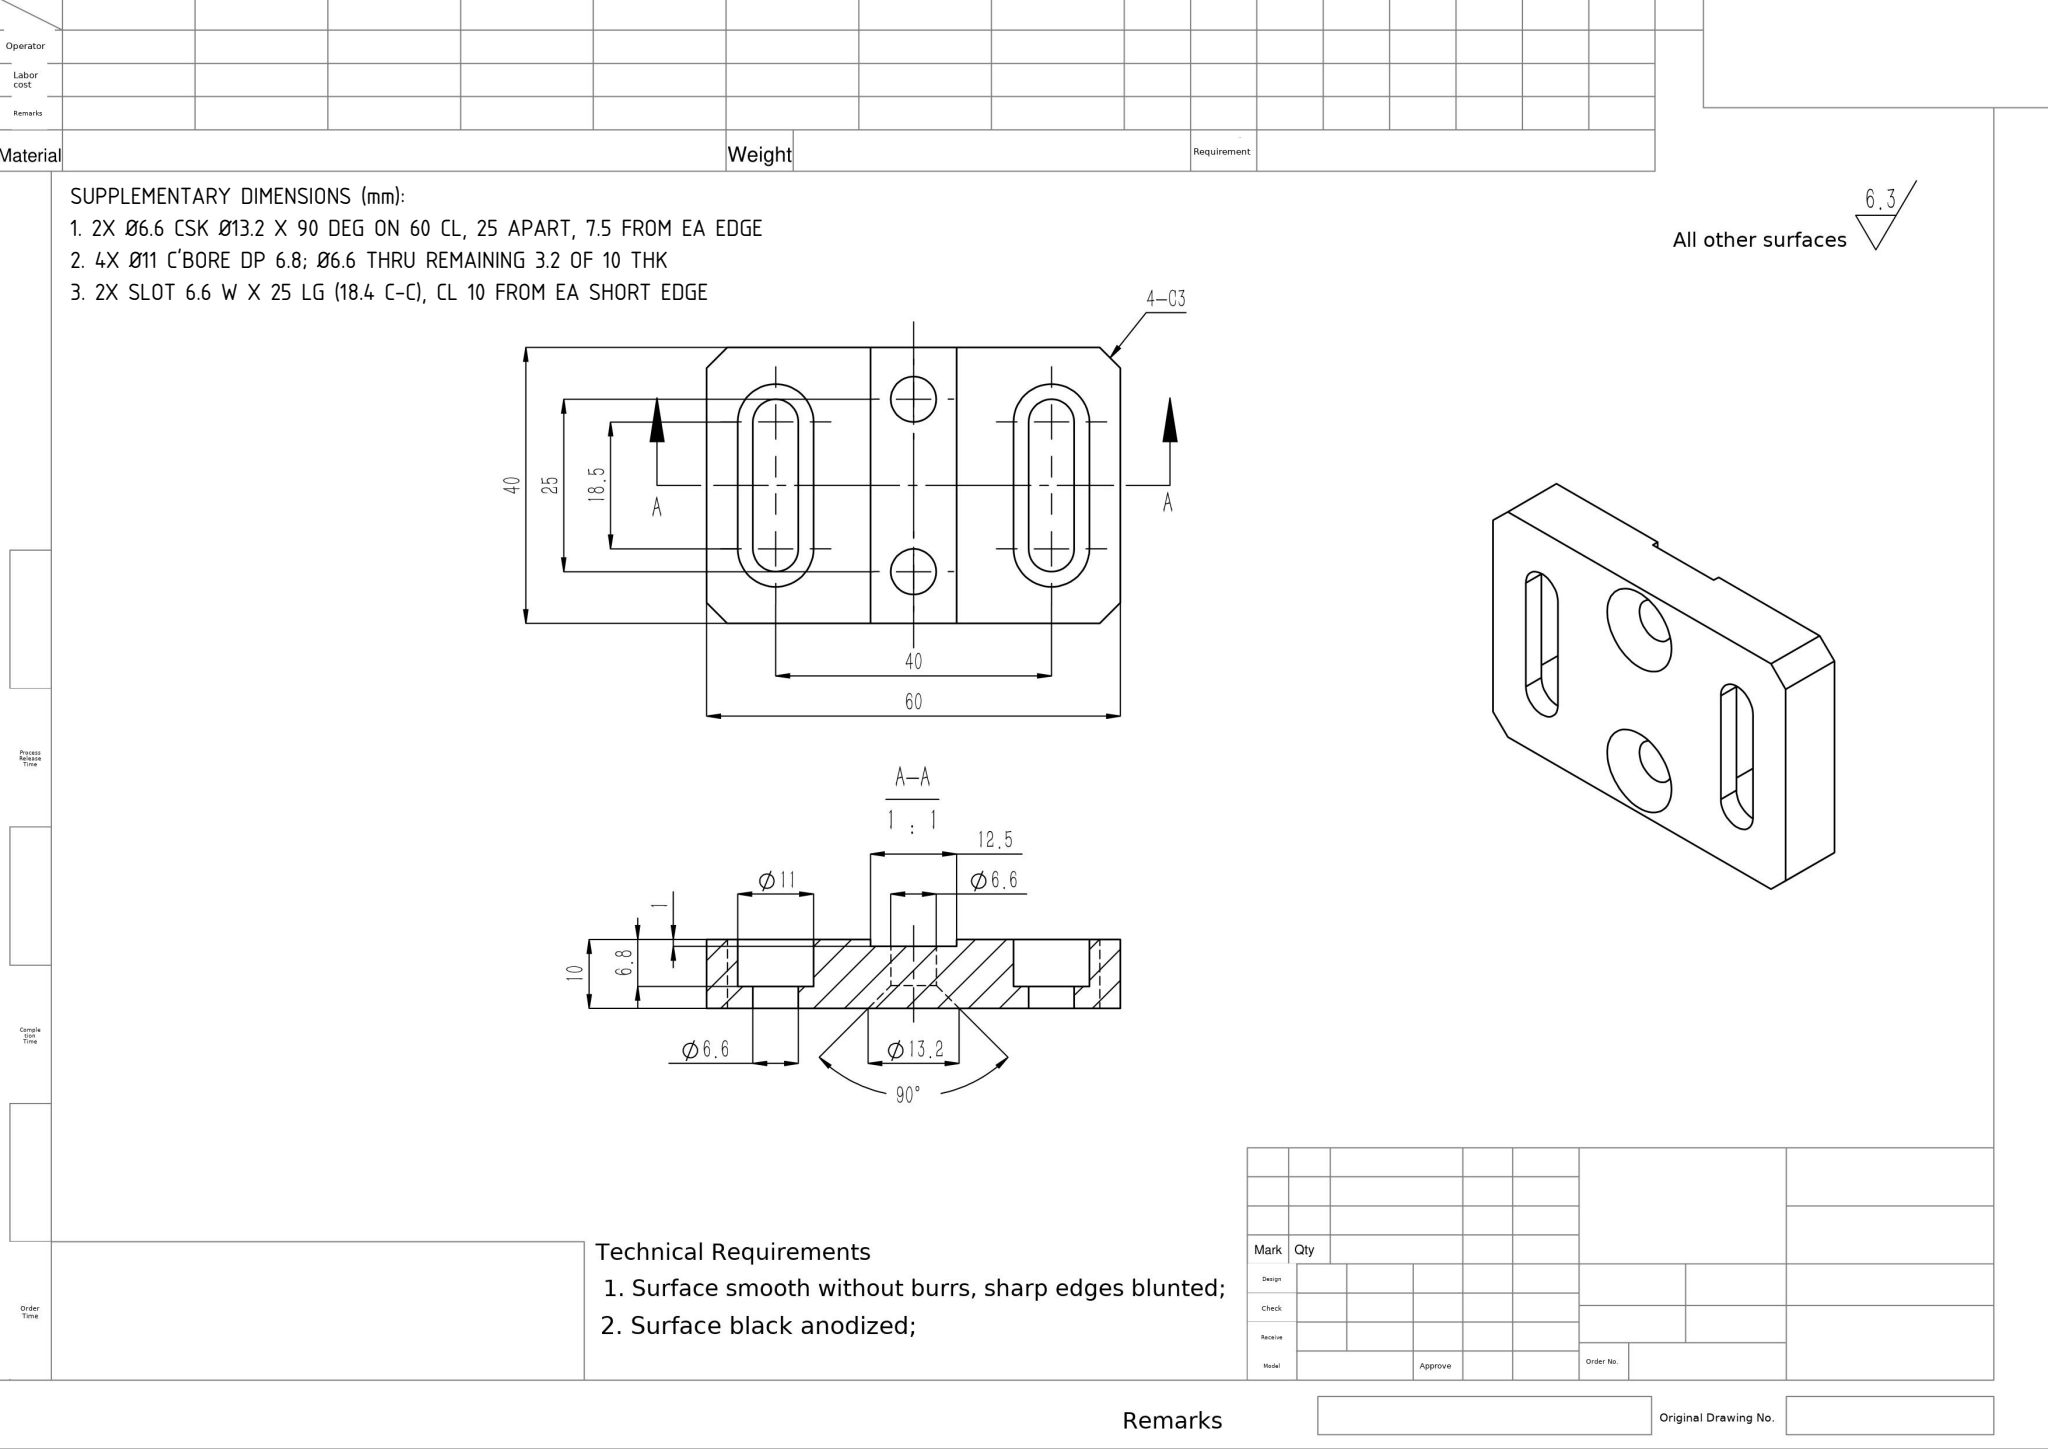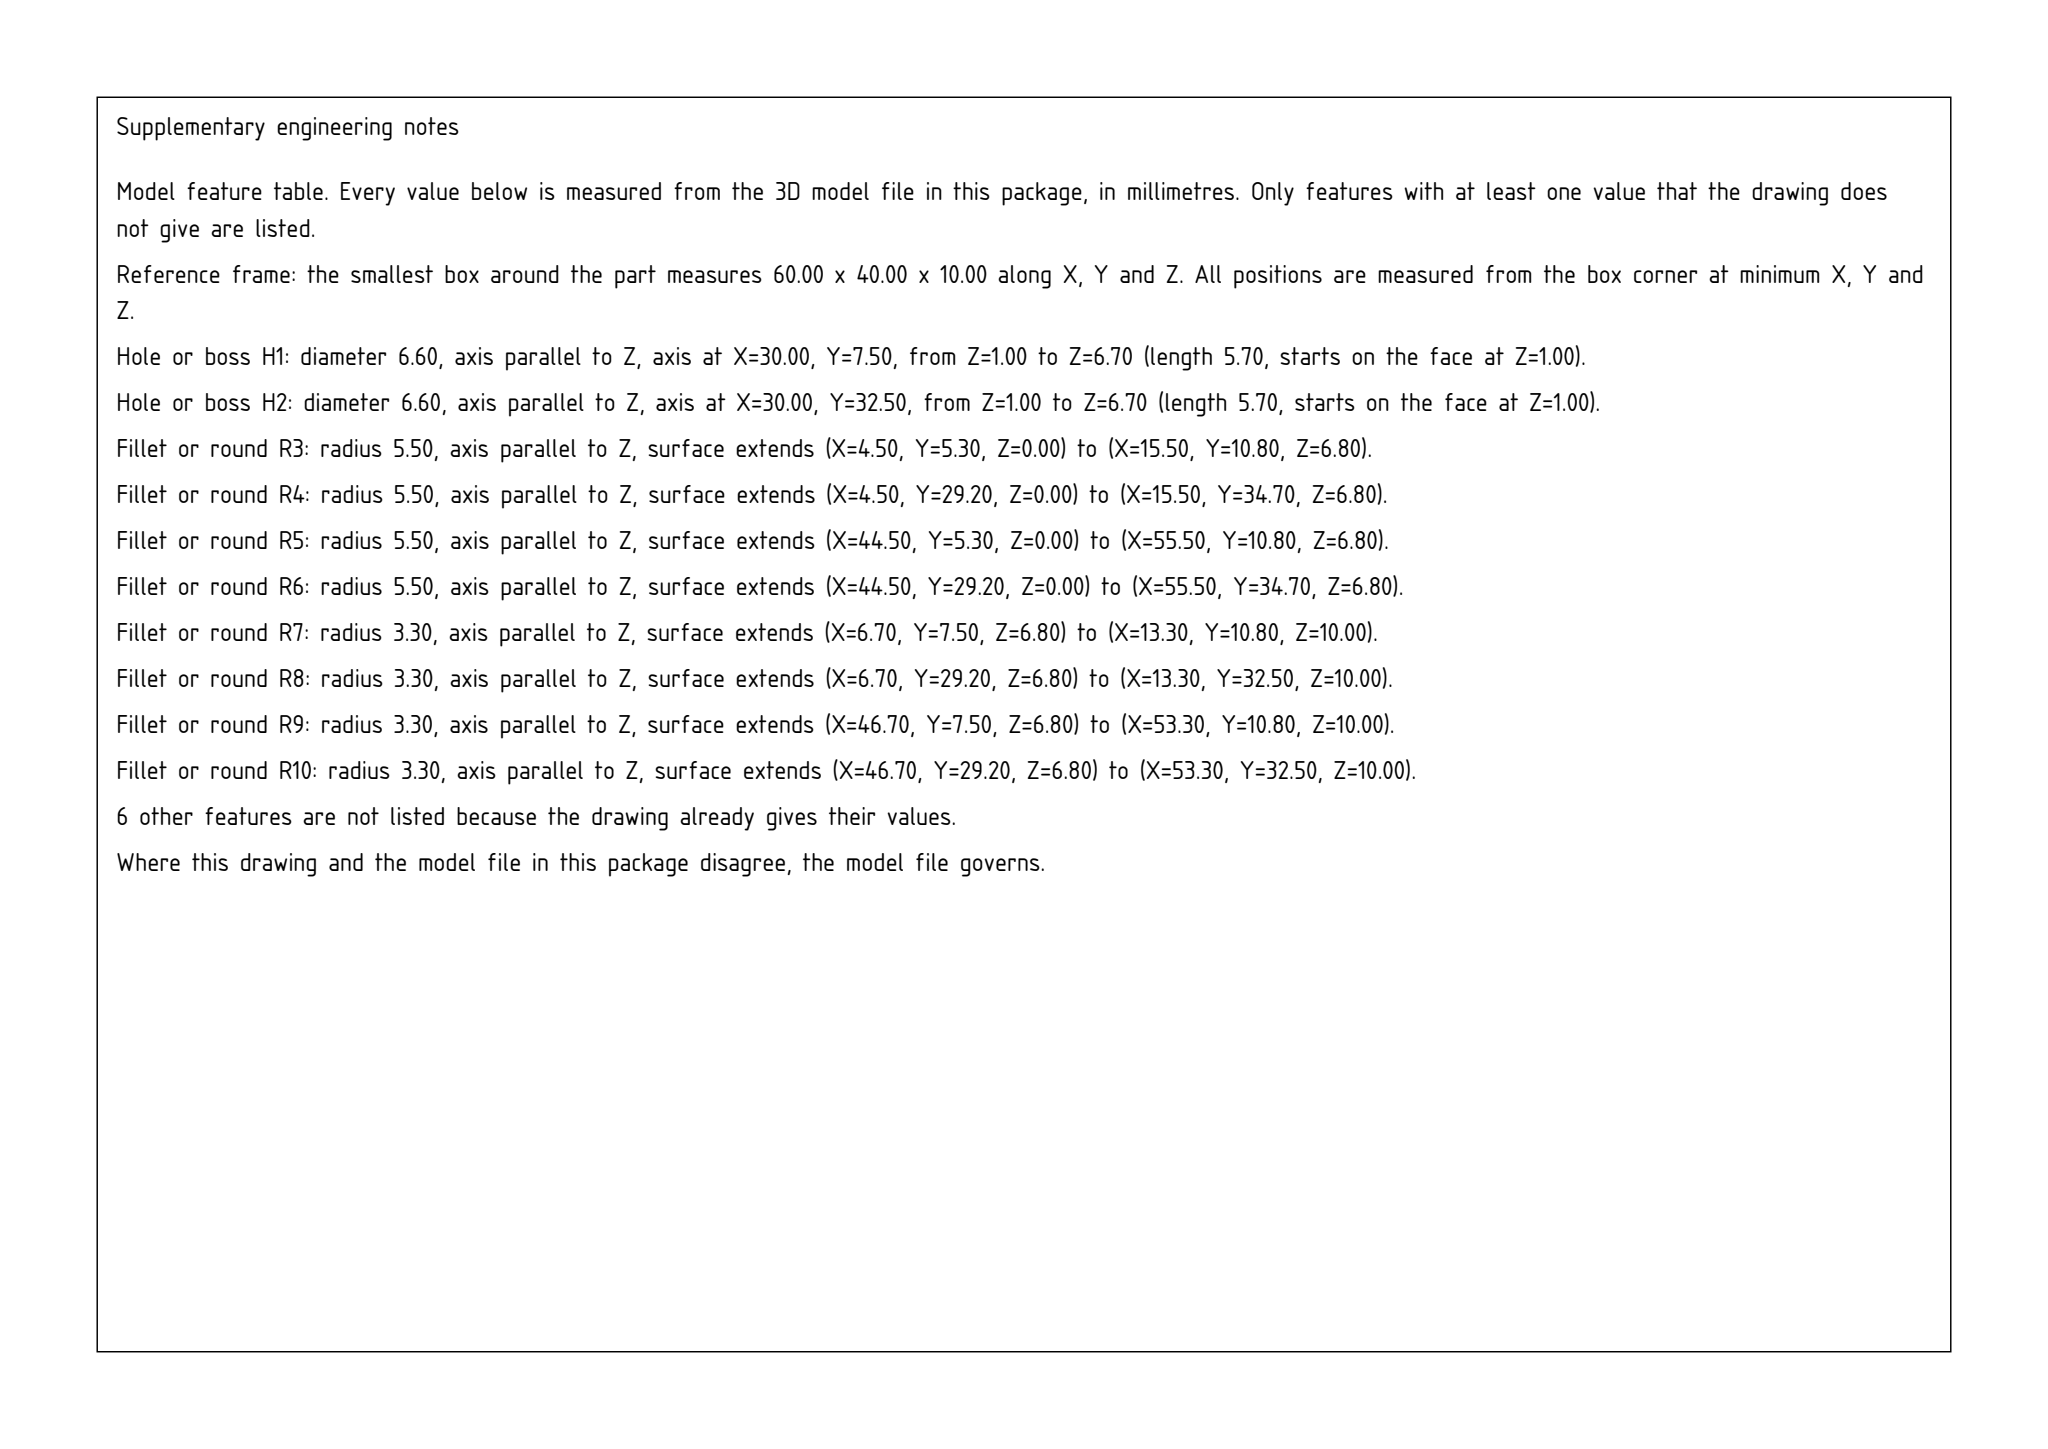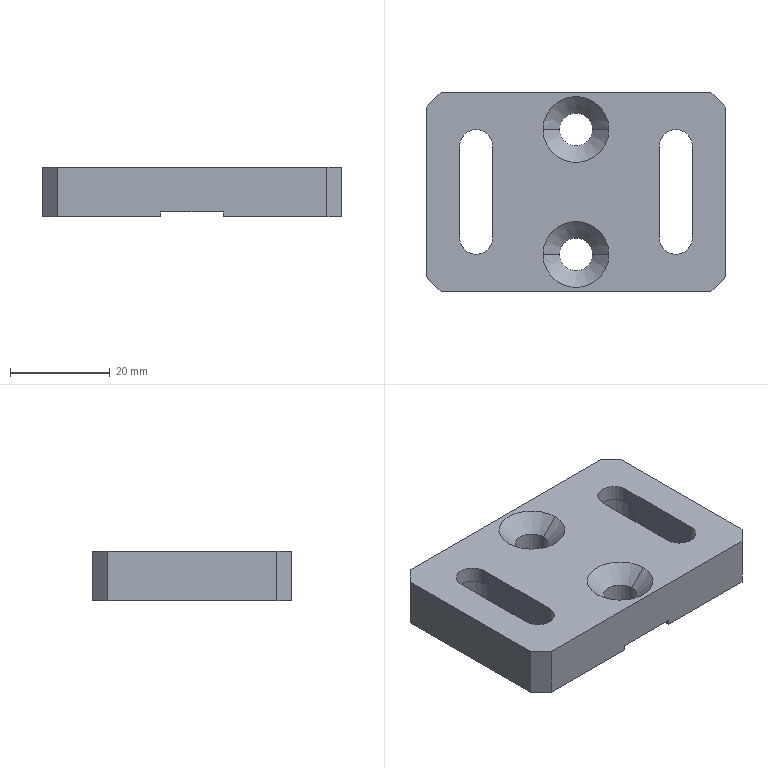Part | SolidWorks | mm | 1 solid | 40 faces | box 60 x 40 x 10 mm | volume 17362 mm3 | plane 24 | cylinder 12 | cone 4 | commonest cylinder face diameters 6.6 x8 11 x4